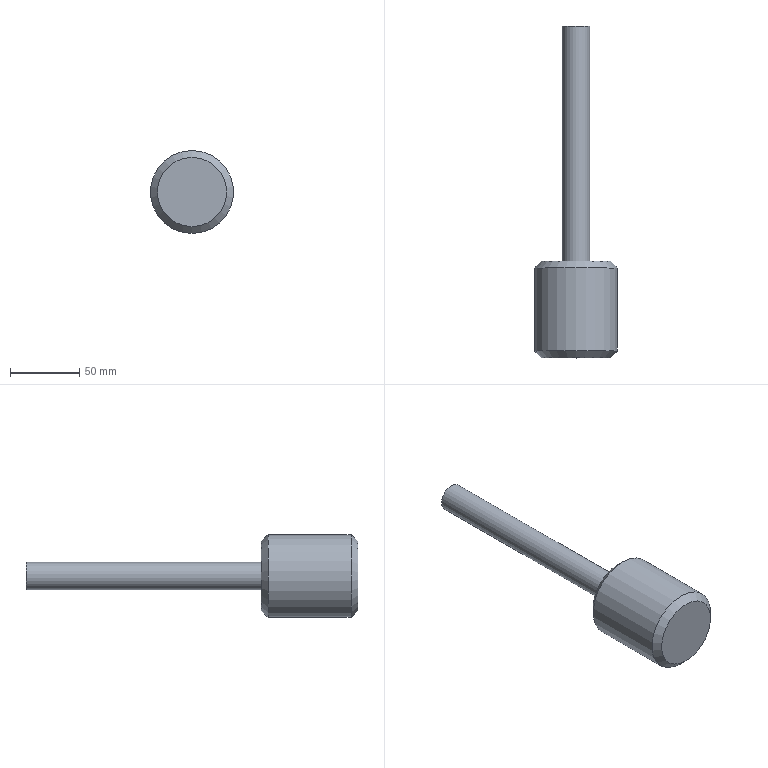Component | NX | EJECTOR2 | 1 solid | 7 faces | box 60 x 240 x 60 mm | volume 246877 mm3 | plane 3 | cylinder 2 | cone 2 | commonest cylinder face diameters 20 x1 60 x1
STEP:
#1=CARTESIAN_POINT('',(0.,0.,0.));
#2=DIRECTION('',(0.,0.,1.));
#3=DIRECTION('',(1.,0.,0.));
#4=AXIS2_PLACEMENT_3D('',#1,#2,#3);
#5=CARTESIAN_POINT('',(0.,55.,-10.));
#6=VERTEX_POINT('',#5);
#7=CARTESIAN_POINT('',(0.,55.,0.));
#8=DIRECTION('',(0.,-1.,0.));
#9=DIRECTION('',(0.,0.,-1.));
#10=AXIS2_PLACEMENT_3D('',#7,#8,#9);
#11=CIRCLE('',#10,10.);
#12=CARTESIAN_POINT('',(0.,55.,0.));
#13=DIRECTION('',(0.,1.,0.));
#14=DIRECTION('',(0.,0.,1.));
#15=AXIS2_PLACEMENT_3D('',#12,#13,#14);
#16=PLANE('',#15);
#17=CARTESIAN_POINT('',(-10.,0.));
#18=CARTESIAN_POINT('',(-10.,17.321));
#19=CARTESIAN_POINT('',(5.,8.66));
#20=CARTESIAN_POINT('',(20.,0.));
#21=CARTESIAN_POINT('',(5.,-8.66));
#22=CARTESIAN_POINT('',(-10.,-17.321));
#23=CARTESIAN_POINT('',(-10.,0.));
#24=(BOUNDED_CURVE()B_SPLINE_CURVE(2,(#17,#18,#19,#20,#21,#22,#23),.UNSPECIFIED.,.T.,.F.)B_SPLINE_CURVE_WITH_KNOTS((1,2,2,2,2,1),(-2.094,0.,2.094,4.189,6.283,8.378),.UNSPECIFIED.)CURVE()GEOMETRIC_REPRESENTATION_ITEM()RATIONAL_B_SPLINE_CURVE((1.,0.5,1.,0.5,1.,0.5,1.))REPRESENTATION_ITEM(''));
#25=(GEOMETRIC_REPRESENTATION_CONTEXT(2)PARAMETRIC_REPRESENTATION_CONTEXT()REPRESENTATION_CONTEXT('',''));
#26=DEFINITIONAL_REPRESENTATION('',(#24),#25);
#27=PCURVE('',#16,#26);
#28=CARTESIAN_POINT('',(0.,55.,0.));
#29=DIRECTION('',(0.,-1.,0.));
#30=DIRECTION('',(0.,0.,-1.));
#31=AXIS2_PLACEMENT_3D('',#28,#29,#30);
#32=CYLINDRICAL_SURFACE('',#31,10.);
#33=CARTESIAN_POINT('',(0.,0.));
#34=DIRECTION('',(1.,0.));
#35=VECTOR('',#34,1.);
#36=LINE('',#33,#35);
#37=(GEOMETRIC_REPRESENTATION_CONTEXT(2)PARAMETRIC_REPRESENTATION_CONTEXT()REPRESENTATION_CONTEXT('',''));
#38=DEFINITIONAL_REPRESENTATION('',(#36),#37);
#39=PCURVE('',#32,#38);
#40=SURFACE_CURVE('',#11,(#27,#39),.PCURVE_S1.);
#41=EDGE_CURVE('',#6,#6,#40,.T.);
#42=ORIENTED_EDGE('',*,*,#41,.F.);
#43=EDGE_LOOP('',(#42));
#44=FACE_BOUND('',#43,.T.);
#45=ADVANCED_FACE('',(#44),#16,.T.);
#46=CARTESIAN_POINT('',(0.,-115.,-10.));
#47=VERTEX_POINT('',#46);
#48=CARTESIAN_POINT('',(0.,-115.,0.));
#49=DIRECTION('',(0.,1.,0.));
#50=DIRECTION('',(0.,0.,-1.));
#51=AXIS2_PLACEMENT_3D('',#48,#49,#50);
#52=CIRCLE('',#51,10.);
#53=CARTESIAN_POINT('',(6.283,170.));
#54=DIRECTION('',(-1.,0.));
#55=VECTOR('',#54,1.);
#56=LINE('',#53,#55);
#57=(GEOMETRIC_REPRESENTATION_CONTEXT(2)PARAMETRIC_REPRESENTATION_CONTEXT()REPRESENTATION_CONTEXT('',''));
#58=DEFINITIONAL_REPRESENTATION('',(#56),#57);
#59=PCURVE('',#32,#58);
#60=CARTESIAN_POINT('',(0.,-115.,0.));
#61=DIRECTION('',(0.,-1.,0.));
#62=DIRECTION('',(0.,0.,-1.));
#63=AXIS2_PLACEMENT_3D('',#60,#61,#62);
#64=PLANE('',#63);
#65=CARTESIAN_POINT('',(10.,0.));
#66=CARTESIAN_POINT('',(10.,-17.321));
#67=CARTESIAN_POINT('',(-5.,-8.66));
#68=CARTESIAN_POINT('',(-20.,-0.));
#69=CARTESIAN_POINT('',(-5.,8.66));
#70=CARTESIAN_POINT('',(10.,17.321));
#71=CARTESIAN_POINT('',(10.,0.));
#72=(BOUNDED_CURVE()B_SPLINE_CURVE(2,(#65,#66,#67,#68,#69,#70,#71),.UNSPECIFIED.,.T.,.F.)B_SPLINE_CURVE_WITH_KNOTS((1,2,2,2,2,1),(-2.094,0.,2.094,4.189,6.283,8.378),.UNSPECIFIED.)CURVE()GEOMETRIC_REPRESENTATION_ITEM()RATIONAL_B_SPLINE_CURVE((1.,0.5,1.,0.5,1.,0.5,1.))REPRESENTATION_ITEM(''));
#73=(GEOMETRIC_REPRESENTATION_CONTEXT(2)PARAMETRIC_REPRESENTATION_CONTEXT()REPRESENTATION_CONTEXT('',''));
#74=DEFINITIONAL_REPRESENTATION('',(#72),#73);
#75=PCURVE('',#64,#74);
#76=SURFACE_CURVE('',#52,(#59,#75),.PCURVE_S1.);
#77=EDGE_CURVE('',#47,#47,#76,.T.);
#78=ORIENTED_EDGE('',*,*,#77,.T.);
#79=CARTESIAN_POINT('',(0.,55.,-10.));
#80=CARTESIAN_POINT('',(0.,-115.,-10.));
#81=B_SPLINE_CURVE_WITH_KNOTS('',1,(#79,#80),.UNSPECIFIED.,.F.,.F.,(2,2),(0.,170.),.PIECEWISE_BEZIER_KNOTS.);
#82=CARTESIAN_POINT('',(0.,0.));
#83=DIRECTION('',(0.,1.));
#84=VECTOR('',#83,1.);
#85=LINE('',#82,#84);
#86=(GEOMETRIC_REPRESENTATION_CONTEXT(2)PARAMETRIC_REPRESENTATION_CONTEXT()REPRESENTATION_CONTEXT('',''));
#87=DEFINITIONAL_REPRESENTATION('',(#85),#86);
#88=PCURVE('',#32,#87);
#89=CARTESIAN_POINT('',(6.283,0.));
#90=DIRECTION('',(0.,1.));
#91=VECTOR('',#90,1.);
#92=LINE('',#89,#91);
#93=(GEOMETRIC_REPRESENTATION_CONTEXT(2)PARAMETRIC_REPRESENTATION_CONTEXT()REPRESENTATION_CONTEXT('',''));
#94=DEFINITIONAL_REPRESENTATION('',(#92),#93);
#95=PCURVE('',#32,#94);
#96=SEAM_CURVE('',#81,(#88,#95),.PCURVE_S1.);
#97=EDGE_CURVE('',#6,#47,#96,.T.);
#98=ORIENTED_EDGE('',*,*,#97,.F.);
#99=ORIENTED_EDGE('',*,*,#41,.T.);
#100=ORIENTED_EDGE('',*,*,#97,.T.);
#101=EDGE_LOOP('',(#78,#98,#99,#100));
#102=FACE_BOUND('',#101,.T.);
#103=ADVANCED_FACE('',(#102),#32,.T.);
#104=CARTESIAN_POINT('',(0.,-120.,-30.));
#105=VERTEX_POINT('',#104);
#106=CARTESIAN_POINT('',(0.,-120.,0.));
#107=DIRECTION('',(0.,-1.,0.));
#108=DIRECTION('',(0.,0.,-1.));
#109=AXIS2_PLACEMENT_3D('',#106,#107,#108);
#110=CIRCLE('',#109,30.);
#111=CARTESIAN_POINT('',(0.,-185.,0.));
#112=DIRECTION('',(0.,1.,0.));
#113=DIRECTION('',(0.,0.,1.));
#114=AXIS2_PLACEMENT_3D('',#111,#112,#113);
#115=CYLINDRICAL_SURFACE('',#114,30.);
#116=CARTESIAN_POINT('',(9.425,65.));
#117=DIRECTION('',(-1.,0.));
#118=VECTOR('',#117,1.);
#119=LINE('',#116,#118);
#120=(GEOMETRIC_REPRESENTATION_CONTEXT(2)PARAMETRIC_REPRESENTATION_CONTEXT()REPRESENTATION_CONTEXT('',''));
#121=DEFINITIONAL_REPRESENTATION('',(#119),#120);
#122=PCURVE('',#115,#121);
#123=CARTESIAN_POINT('',(0.,-120.,0.));
#124=DIRECTION('',(0.,-1.,0.));
#125=DIRECTION('',(0.,0.,-1.));
#126=AXIS2_PLACEMENT_3D('',#123,#124,#125);
#127=CONICAL_SURFACE('',#126,30.,0.7854);
#128=CARTESIAN_POINT('',(0.,0.));
#129=DIRECTION('',(1.,0.));
#130=VECTOR('',#129,1.);
#131=LINE('',#128,#130);
#132=(GEOMETRIC_REPRESENTATION_CONTEXT(2)PARAMETRIC_REPRESENTATION_CONTEXT()REPRESENTATION_CONTEXT('',''));
#133=DEFINITIONAL_REPRESENTATION('',(#131),#132);
#134=PCURVE('',#127,#133);
#135=SURFACE_CURVE('',#110,(#122,#134),.PCURVE_S1.);
#136=EDGE_CURVE('',#105,#105,#135,.T.);
#137=ORIENTED_EDGE('',*,*,#136,.T.);
#138=CARTESIAN_POINT('',(0.,-180.,-30.));
#139=VERTEX_POINT('',#138);
#140=CARTESIAN_POINT('',(0.,-180.,-30.));
#141=CARTESIAN_POINT('',(0.,-120.,-30.));
#142=B_SPLINE_CURVE_WITH_KNOTS('',1,(#140,#141),.UNSPECIFIED.,.F.,.F.,(2,2),(5.,65.),.PIECEWISE_BEZIER_KNOTS.);
#143=CARTESIAN_POINT('',(3.142,0.));
#144=DIRECTION('',(0.,1.));
#145=VECTOR('',#144,1.);
#146=LINE('',#143,#145);
#147=(GEOMETRIC_REPRESENTATION_CONTEXT(2)PARAMETRIC_REPRESENTATION_CONTEXT()REPRESENTATION_CONTEXT('',''));
#148=DEFINITIONAL_REPRESENTATION('',(#146),#147);
#149=PCURVE('',#115,#148);
#150=CARTESIAN_POINT('',(9.425,0.));
#151=DIRECTION('',(0.,1.));
#152=VECTOR('',#151,1.);
#153=LINE('',#150,#152);
#154=(GEOMETRIC_REPRESENTATION_CONTEXT(2)PARAMETRIC_REPRESENTATION_CONTEXT()REPRESENTATION_CONTEXT('',''));
#155=DEFINITIONAL_REPRESENTATION('',(#153),#154);
#156=PCURVE('',#115,#155);
#157=SEAM_CURVE('',#142,(#149,#156),.PCURVE_S1.);
#158=EDGE_CURVE('',#139,#105,#157,.T.);
#159=ORIENTED_EDGE('',*,*,#158,.F.);
#160=CARTESIAN_POINT('',(0.,-180.,0.));
#161=DIRECTION('',(0.,1.,0.));
#162=DIRECTION('',(0.,0.,-1.));
#163=AXIS2_PLACEMENT_3D('',#160,#161,#162);
#164=CIRCLE('',#163,30.);
#165=CARTESIAN_POINT('',(3.142,5.));
#166=DIRECTION('',(1.,0.));
#167=VECTOR('',#166,1.);
#168=LINE('',#165,#167);
#169=(GEOMETRIC_REPRESENTATION_CONTEXT(2)PARAMETRIC_REPRESENTATION_CONTEXT()REPRESENTATION_CONTEXT('',''));
#170=DEFINITIONAL_REPRESENTATION('',(#168),#169);
#171=PCURVE('',#115,#170);
#172=CARTESIAN_POINT('',(0.,-185.,0.));
#173=DIRECTION('',(0.,1.,0.));
#174=DIRECTION('',(0.,0.,1.));
#175=AXIS2_PLACEMENT_3D('',#172,#173,#174);
#176=CONICAL_SURFACE('',#175,25.,0.7854);
#177=CARTESIAN_POINT('',(3.142,5.));
#178=DIRECTION('',(1.,0.));
#179=VECTOR('',#178,1.);
#180=LINE('',#177,#179);
#181=(GEOMETRIC_REPRESENTATION_CONTEXT(2)PARAMETRIC_REPRESENTATION_CONTEXT()REPRESENTATION_CONTEXT('',''));
#182=DEFINITIONAL_REPRESENTATION('',(#180),#181);
#183=PCURVE('',#176,#182);
#184=SURFACE_CURVE('',#164,(#171,#183),.PCURVE_S1.);
#185=EDGE_CURVE('',#139,#139,#184,.T.);
#186=ORIENTED_EDGE('',*,*,#185,.T.);
#187=ORIENTED_EDGE('',*,*,#158,.T.);
#188=EDGE_LOOP('',(#137,#159,#186,#187));
#189=FACE_BOUND('',#188,.T.);
#190=ADVANCED_FACE('',(#189),#115,.T.);
#191=CARTESIAN_POINT('',(0.,-185.,-25.));
#192=VERTEX_POINT('',#191);
#193=CARTESIAN_POINT('',(0.,-185.,0.));
#194=DIRECTION('',(0.,-1.,0.));
#195=DIRECTION('',(0.,0.,-1.));
#196=AXIS2_PLACEMENT_3D('',#193,#194,#195);
#197=CIRCLE('',#196,25.);
#198=CARTESIAN_POINT('',(0.,-185.,0.));
#199=DIRECTION('',(0.,-1.,0.));
#200=DIRECTION('',(0.,0.,-1.));
#201=AXIS2_PLACEMENT_3D('',#198,#199,#200);
#202=PLANE('',#201);
#203=CARTESIAN_POINT('',(0.,0.));
#204=DIRECTION('',(1.,0.));
#205=AXIS2_PLACEMENT_2D('',#203,#204);
#206=CIRCLE('',#205,25.);
#207=(GEOMETRIC_REPRESENTATION_CONTEXT(2)PARAMETRIC_REPRESENTATION_CONTEXT()REPRESENTATION_CONTEXT('',''));
#208=DEFINITIONAL_REPRESENTATION('',(#206),#207);
#209=PCURVE('',#202,#208);
#210=CARTESIAN_POINT('',(9.425,0.));
#211=DIRECTION('',(-1.,0.));
#212=VECTOR('',#211,1.);
#213=LINE('',#210,#212);
#214=(GEOMETRIC_REPRESENTATION_CONTEXT(2)PARAMETRIC_REPRESENTATION_CONTEXT()REPRESENTATION_CONTEXT('',''));
#215=DEFINITIONAL_REPRESENTATION('',(#213),#214);
#216=PCURVE('',#176,#215);
#217=SURFACE_CURVE('',#197,(#209,#216),.PCURVE_S1.);
#218=EDGE_CURVE('',#192,#192,#217,.T.);
#219=ORIENTED_EDGE('',*,*,#218,.T.);
#220=EDGE_LOOP('',(#219));
#221=FACE_BOUND('',#220,.T.);
#222=ADVANCED_FACE('',(#221),#202,.T.);
#223=CARTESIAN_POINT('',(0.,-115.,-25.));
#224=VERTEX_POINT('',#223);
#225=CARTESIAN_POINT('',(0.,-115.,0.));
#226=DIRECTION('',(0.,1.,0.));
#227=DIRECTION('',(0.,0.,-1.));
#228=AXIS2_PLACEMENT_3D('',#225,#226,#227);
#229=CIRCLE('',#228,25.);
#230=CARTESIAN_POINT('',(25.,0.));
#231=CARTESIAN_POINT('',(25.,-43.301));
#232=CARTESIAN_POINT('',(-12.5,-21.651));
#233=CARTESIAN_POINT('',(-50.,-0.));
#234=CARTESIAN_POINT('',(-12.5,21.651));
#235=CARTESIAN_POINT('',(25.,43.301));
#236=CARTESIAN_POINT('',(25.,0.));
#237=(BOUNDED_CURVE()B_SPLINE_CURVE(2,(#230,#231,#232,#233,#234,#235,#236),.UNSPECIFIED.,.T.,.F.)B_SPLINE_CURVE_WITH_KNOTS((1,2,2,2,2,1),(-2.094,0.,2.094,4.189,6.283,8.378),.UNSPECIFIED.)CURVE()GEOMETRIC_REPRESENTATION_ITEM()RATIONAL_B_SPLINE_CURVE((1.,0.5,1.,0.5,1.,0.5,1.))REPRESENTATION_ITEM(''));
#238=(GEOMETRIC_REPRESENTATION_CONTEXT(2)PARAMETRIC_REPRESENTATION_CONTEXT()REPRESENTATION_CONTEXT('',''));
#239=DEFINITIONAL_REPRESENTATION('',(#237),#238);
#240=PCURVE('',#64,#239);
#241=CARTESIAN_POINT('',(6.283,-5.));
#242=DIRECTION('',(-1.,0.));
#243=VECTOR('',#242,1.);
#244=LINE('',#241,#243);
#245=(GEOMETRIC_REPRESENTATION_CONTEXT(2)PARAMETRIC_REPRESENTATION_CONTEXT()REPRESENTATION_CONTEXT('',''));
#246=DEFINITIONAL_REPRESENTATION('',(#244),#245);
#247=PCURVE('',#127,#246);
#248=SURFACE_CURVE('',#229,(#240,#247),.PCURVE_S1.);
#249=EDGE_CURVE('',#224,#224,#248,.T.);
#250=ORIENTED_EDGE('',*,*,#249,.T.);
#251=EDGE_LOOP('',(#250));
#252=FACE_BOUND('',#251,.T.);
#253=ORIENTED_EDGE('',*,*,#77,.F.);
#254=EDGE_LOOP('',(#253));
#255=FACE_BOUND('',#254,.T.);
#256=ADVANCED_FACE('',(#252,#255),#64,.F.);
#257=ORIENTED_EDGE('',*,*,#249,.F.);
#258=CARTESIAN_POINT('',(0.,-115.,-25.));
#259=CARTESIAN_POINT('',(0.,-120.,-30.));
#260=B_SPLINE_CURVE_WITH_KNOTS('',1,(#258,#259),.UNSPECIFIED.,.F.,.F.,(2,2),(-7.071,0.),.PIECEWISE_BEZIER_KNOTS.);
#261=CARTESIAN_POINT('',(6.283,0.));
#262=DIRECTION('',(0.,1.));
#263=VECTOR('',#262,1.);
#264=LINE('',#261,#263);
#265=(GEOMETRIC_REPRESENTATION_CONTEXT(2)PARAMETRIC_REPRESENTATION_CONTEXT()REPRESENTATION_CONTEXT('',''));
#266=DEFINITIONAL_REPRESENTATION('',(#264),#265);
#267=PCURVE('',#127,#266);
#268=CARTESIAN_POINT('',(0.,0.));
#269=DIRECTION('',(0.,1.));
#270=VECTOR('',#269,1.);
#271=LINE('',#268,#270);
#272=(GEOMETRIC_REPRESENTATION_CONTEXT(2)PARAMETRIC_REPRESENTATION_CONTEXT()REPRESENTATION_CONTEXT('',''));
#273=DEFINITIONAL_REPRESENTATION('',(#271),#272);
#274=PCURVE('',#127,#273);
#275=SEAM_CURVE('',#260,(#267,#274),.PCURVE_S1.);
#276=EDGE_CURVE('',#224,#105,#275,.T.);
#277=ORIENTED_EDGE('',*,*,#276,.T.);
#278=ORIENTED_EDGE('',*,*,#136,.F.);
#279=ORIENTED_EDGE('',*,*,#276,.F.);
#280=EDGE_LOOP('',(#257,#277,#278,#279));
#281=FACE_BOUND('',#280,.T.);
#282=ADVANCED_FACE('',(#281),#127,.T.);
#283=ORIENTED_EDGE('',*,*,#185,.F.);
#284=CARTESIAN_POINT('',(0.,-185.,-25.));
#285=CARTESIAN_POINT('',(0.,-180.,-30.));
#286=B_SPLINE_CURVE_WITH_KNOTS('',1,(#284,#285),.UNSPECIFIED.,.F.,.F.,(2,2),(0.,7.071),.PIECEWISE_BEZIER_KNOTS.);
#287=CARTESIAN_POINT('',(3.142,0.));
#288=DIRECTION('',(0.,1.));
#289=VECTOR('',#288,1.);
#290=LINE('',#287,#289);
#291=(GEOMETRIC_REPRESENTATION_CONTEXT(2)PARAMETRIC_REPRESENTATION_CONTEXT()REPRESENTATION_CONTEXT('',''));
#292=DEFINITIONAL_REPRESENTATION('',(#290),#291);
#293=PCURVE('',#176,#292);
#294=CARTESIAN_POINT('',(9.425,0.));
#295=DIRECTION('',(0.,1.));
#296=VECTOR('',#295,1.);
#297=LINE('',#294,#296);
#298=(GEOMETRIC_REPRESENTATION_CONTEXT(2)PARAMETRIC_REPRESENTATION_CONTEXT()REPRESENTATION_CONTEXT('',''));
#299=DEFINITIONAL_REPRESENTATION('',(#297),#298);
#300=PCURVE('',#176,#299);
#301=SEAM_CURVE('',#286,(#293,#300),.PCURVE_S1.);
#302=EDGE_CURVE('',#192,#139,#301,.T.);
#303=ORIENTED_EDGE('',*,*,#302,.F.);
#304=ORIENTED_EDGE('',*,*,#218,.F.);
#305=ORIENTED_EDGE('',*,*,#302,.T.);
#306=EDGE_LOOP('',(#283,#303,#304,#305));
#307=FACE_BOUND('',#306,.T.);
#308=ADVANCED_FACE('',(#307),#176,.T.);
#309=CLOSED_SHELL('',(#45,#103,#190,#222,#256,#282,#308));
#310=MANIFOLD_SOLID_BREP('',#309);
#311=(LENGTH_UNIT()NAMED_UNIT(*)SI_UNIT(.MILLI.,.METRE.));
#312=UNCERTAINTY_MEASURE_WITH_UNIT(LENGTH_MEASURE(0.00001),#311,'','');
#313=(NAMED_UNIT(*)PLANE_ANGLE_UNIT()SI_UNIT($,.RADIAN.));
#314=(NAMED_UNIT(*)SI_UNIT($,.STERADIAN.)SOLID_ANGLE_UNIT());
#315=(GEOMETRIC_REPRESENTATION_CONTEXT(3)GLOBAL_UNCERTAINTY_ASSIGNED_CONTEXT((#312))GLOBAL_UNIT_ASSIGNED_CONTEXT((#311,#313,#314))REPRESENTATION_CONTEXT('',''));
#316=ADVANCED_BREP_SHAPE_REPRESENTATION('',(#4,#310),#315);